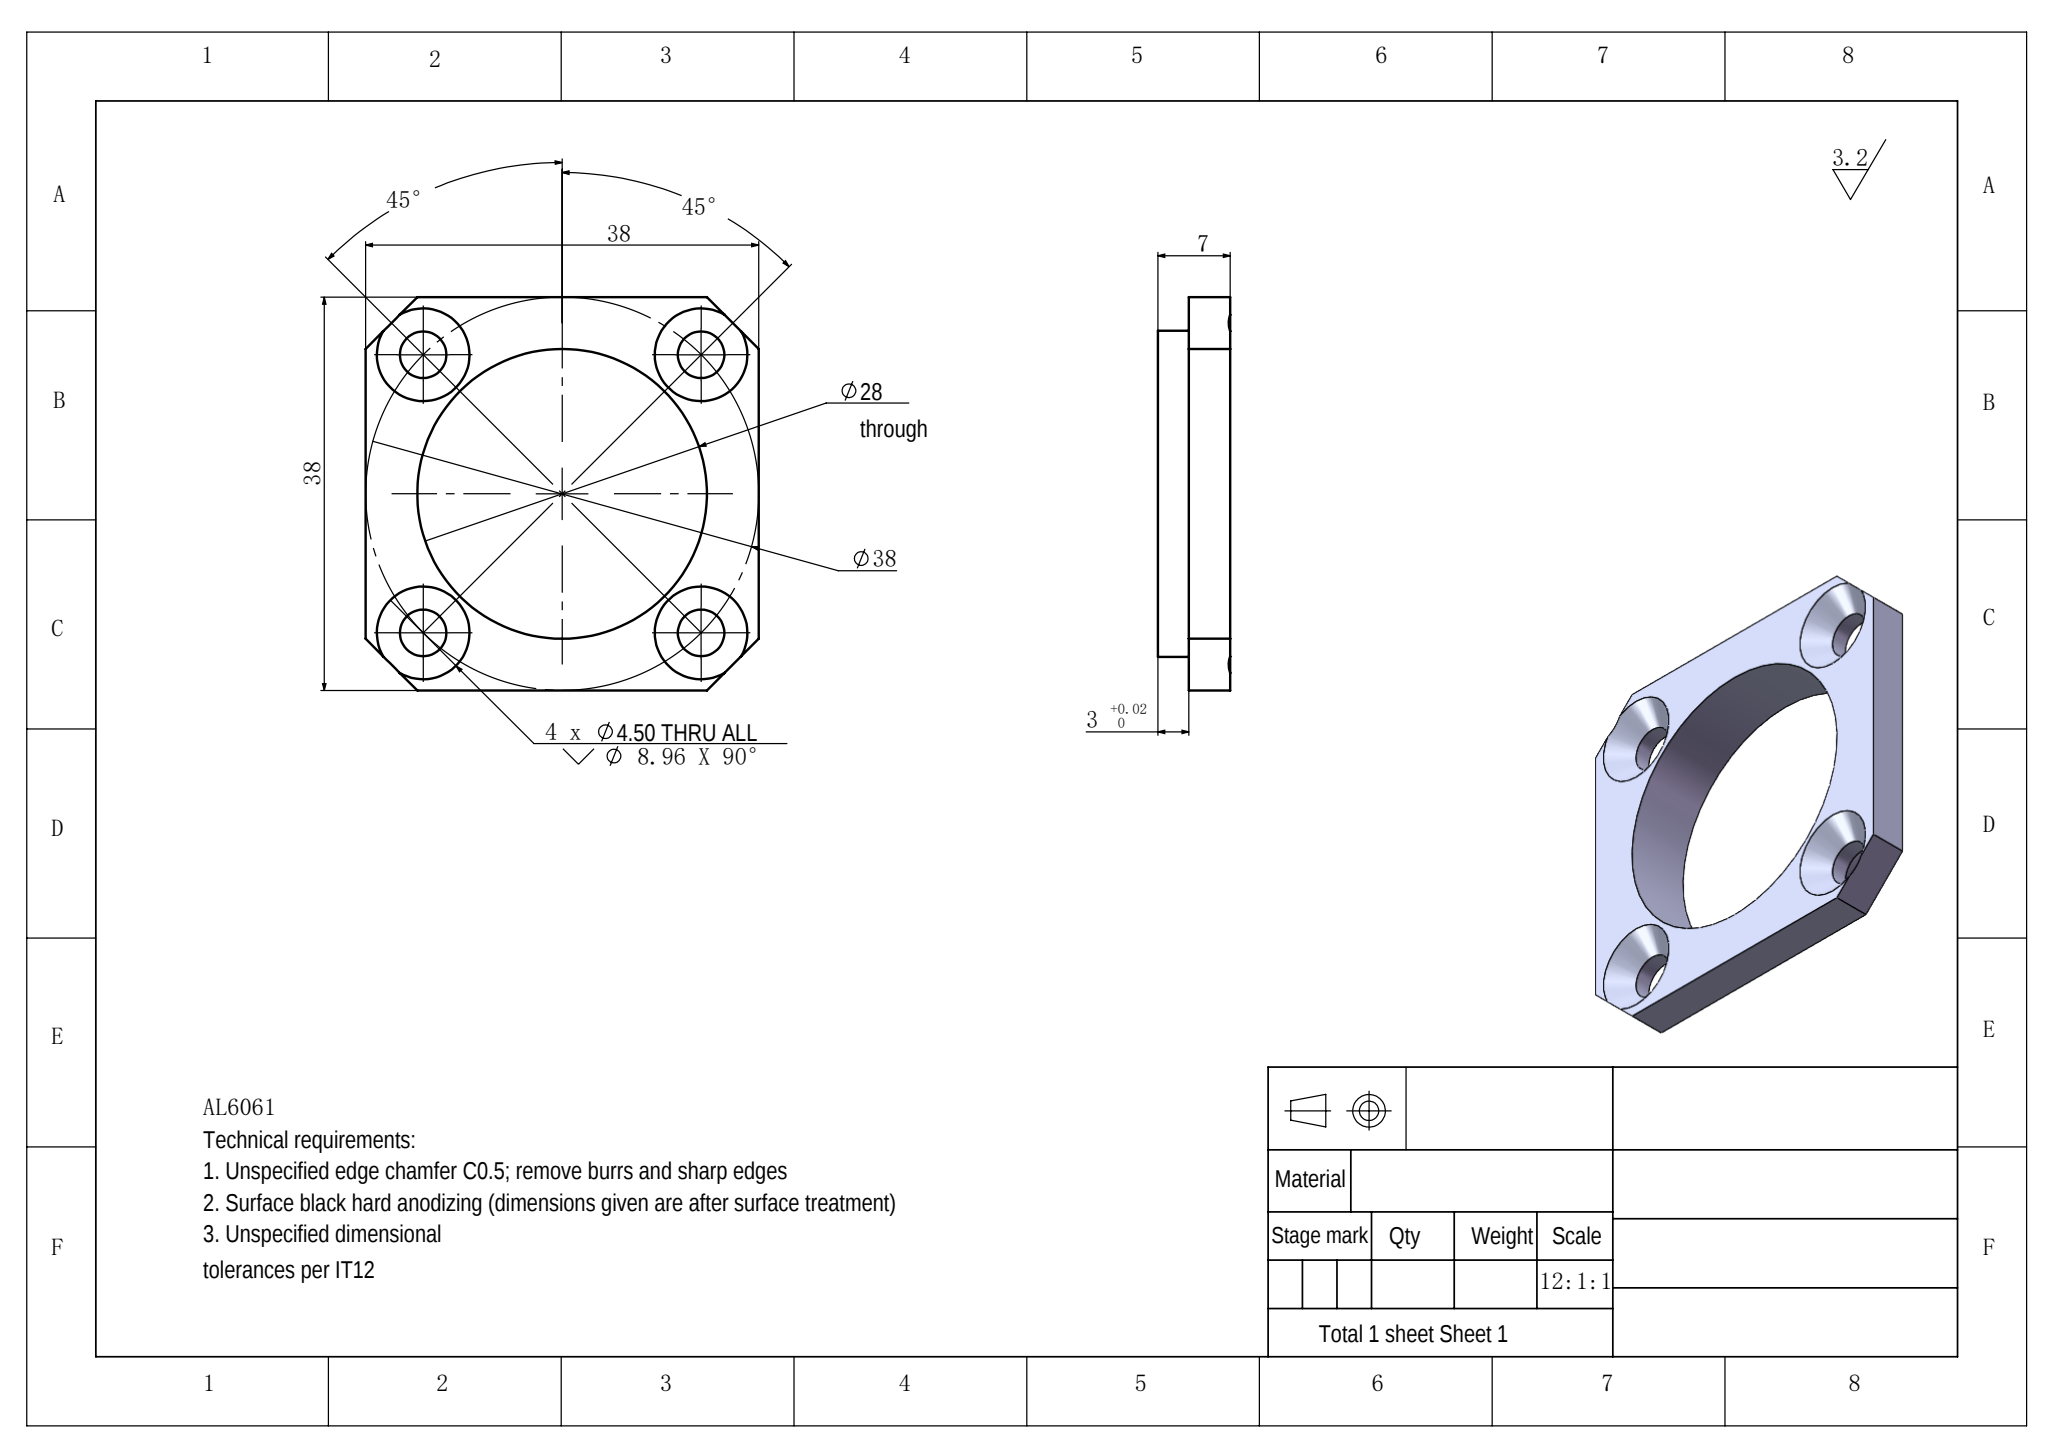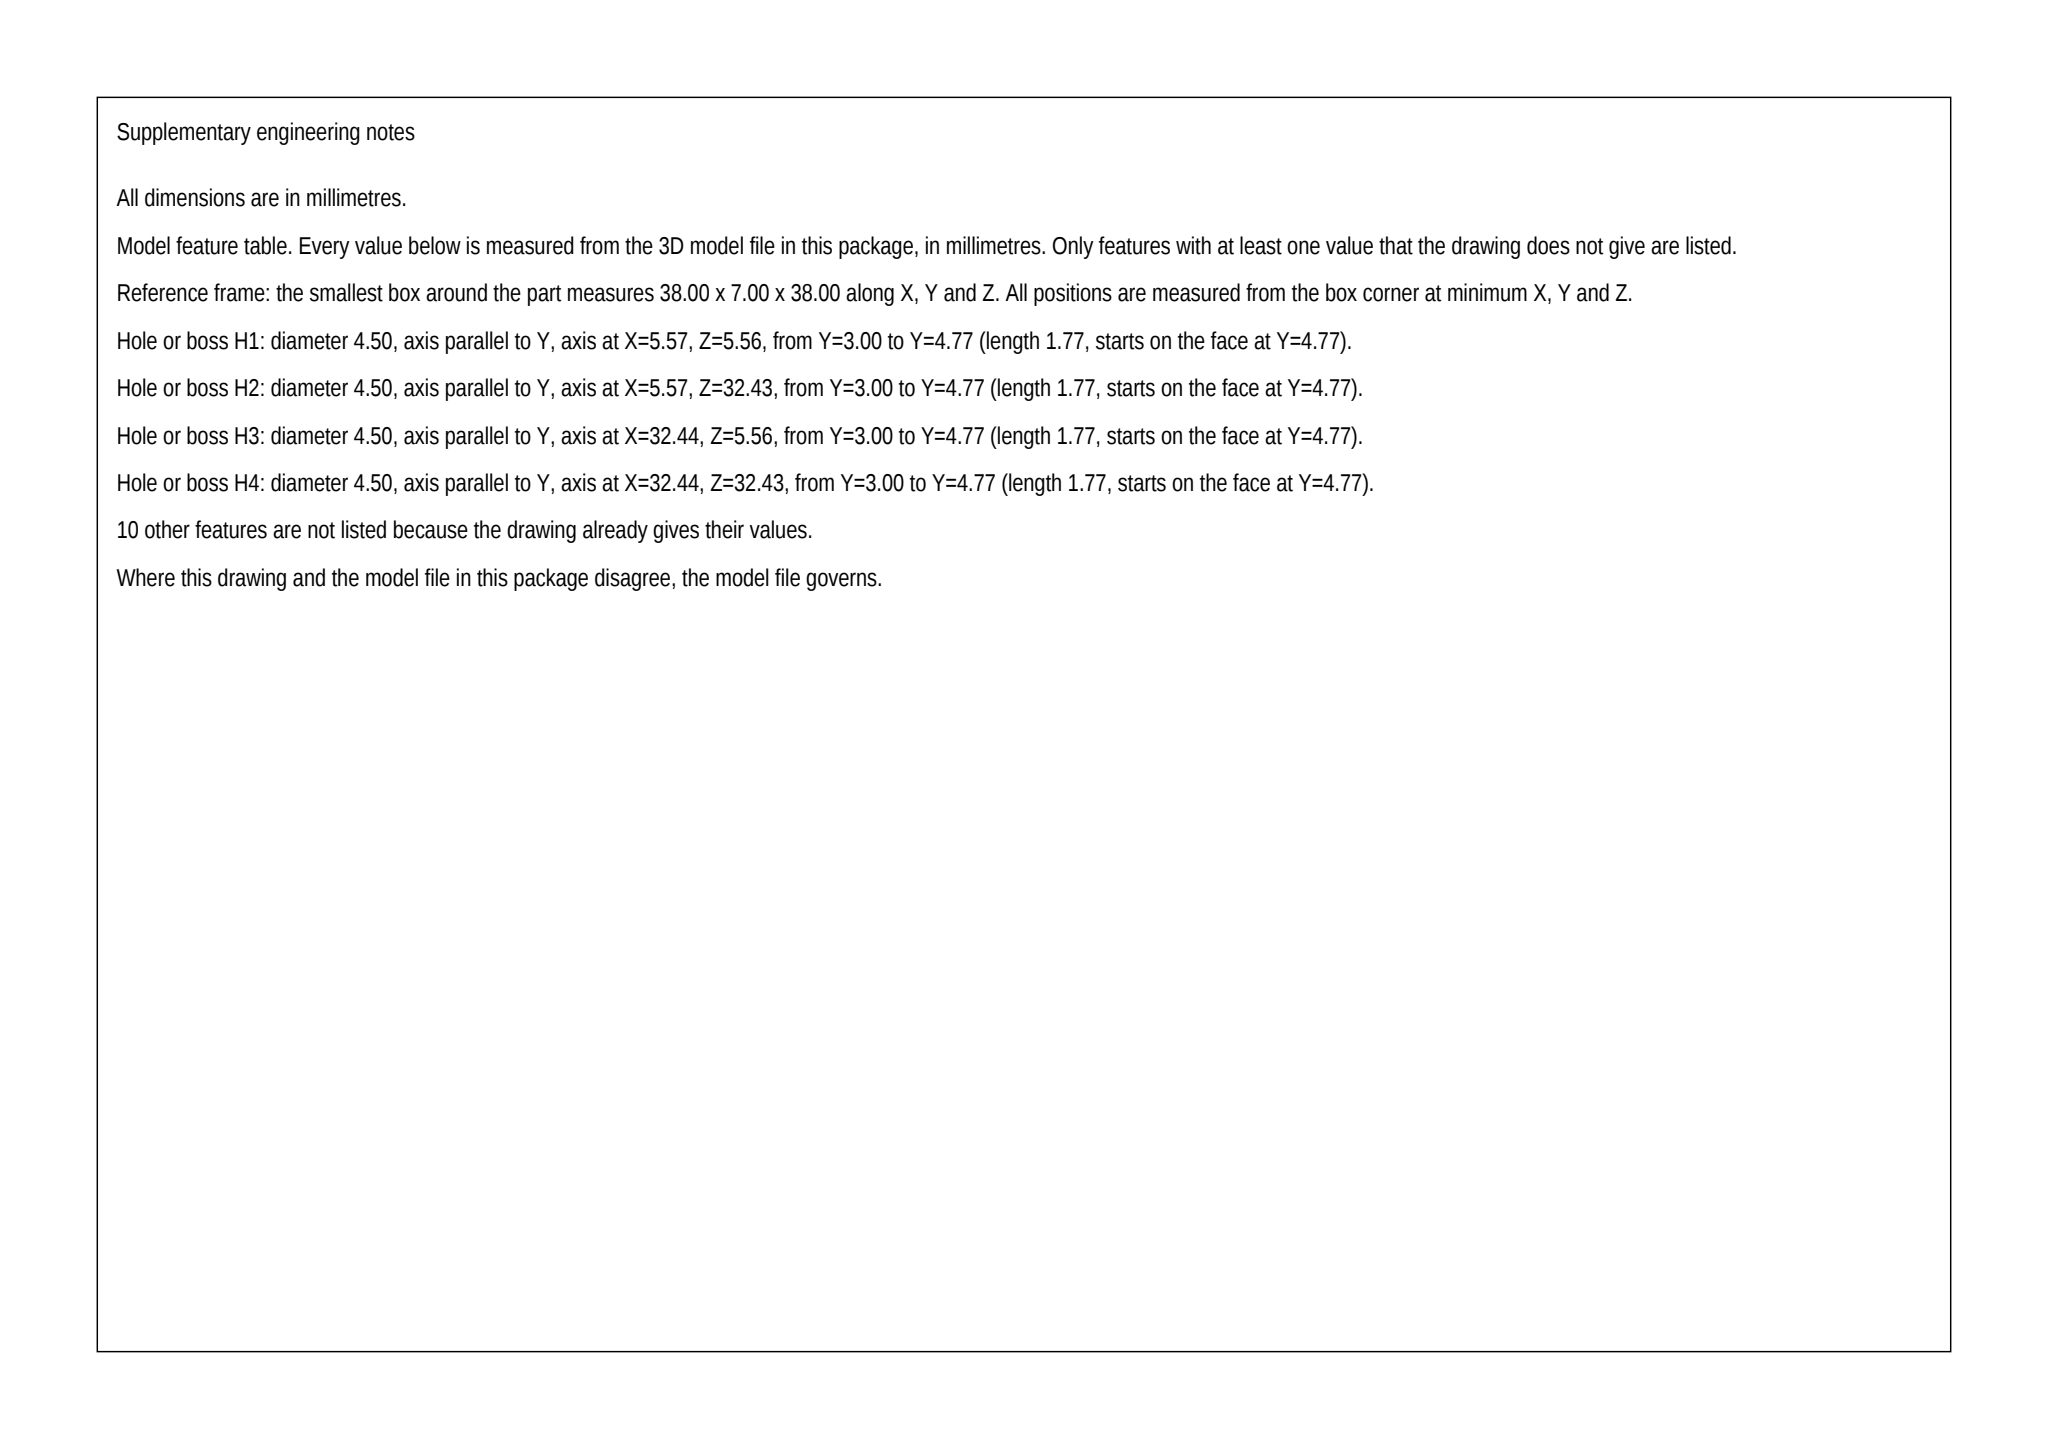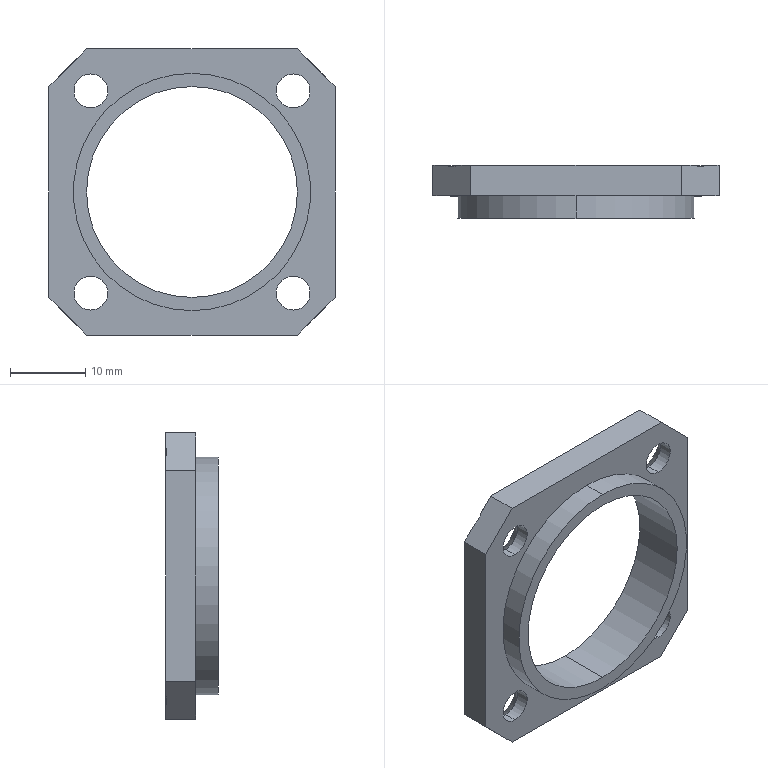Part | SolidWorks | mm | material AL6061 | 1 solid | 31 faces | box 38 x 7 x 38 mm | volume 3162 mm3 | cylinder 12 | plane 11 | cone 8 | commonest cylinder face diameters 4.5 x8 31.5 x2 28 x2
build123d program:
from build123d import *
from build123d.topology import SkipClean

# Parameters (mm, degrees)
SKETCH1_R                                    = 14
EXTRUDE1_DEPTH                               = 4
M4_HEX_SOCKET_COUNTERSUNK_HEAD_SCREW_2_COUNT = 2
M4_HEX_SOCKET_COUNTERSUNK_HEAD_SCREW_2_PITCH = 26.87
M4_HEX_SOCKET_COUNTERSUNK_HEAD_SCREW_3_COUNT = 2
M4_HEX_SOCKET_COUNTERSUNK_HEAD_SCREW_3_PITCH = 26.87
M4_HEX_SOCKET_COUNTERSUNK_HEAD_SCREW_4_COUNT = 2
M4_HEX_SOCKET_COUNTERSUNK_HEAD_SCREW_4_PITCH = 38
BOSS_EXTRUDE1_START                          = 3
SKETCH4_R                                    = 15.75
SKETCH4_R_2                                  = 14
BOSS_EXTRUDE1_DEPTH                          = 3


with BuildPart() as part:
    # Sketch1 → Extrude1 (new body)
    with BuildSketch(Plane(origin=(0, 0, 0), x_dir=(1, 0, 0), z_dir=(0, 1, 0))):
        Polygon((-81.535, -12.039), (-76.535, -7.039), (-48.535, -7.039), (-43.535, -12.039), (-43.535, -40.039), (-48.535, -45.039), (-76.535, -45.039), (-81.535, -40.039), align=None)
        with Locations(Location((-62.535, -26.039, 0), (0, 0, 270))):
            Circle(SKETCH1_R, mode=Mode.SUBTRACT)
    extrude(amount=EXTRUDE1_DEPTH)

    # Sketch3 → M4 Hex Socket Countersunk Head Screw Cou (revolve, cut)
    with BuildSketch(Plane(origin=(-75.97, 4, 12.604), x_dir=(0, 0, 1), z_dir=(1, 0, 0))):
        Polygon((0, 0), (0, 4), (2.25, 4), (2.25, 2.23), (4.48, 0), align=None)
    m4_hex_socket_countersunk_head_screw_cou = revolve(axis=Axis((-75.97, 10.35, 12.604), (0, -1, 0)), mode=Mode.SUBTRACT)

    # M4 Hex Socket Countersunk Head Screw 2: M4 Hex Socket Countersunk Head Screw Cou ×2
    with Locations(*[(i * M4_HEX_SOCKET_COUNTERSUNK_HEAD_SCREW_2_PITCH, 0, 0) for i in range(1, M4_HEX_SOCKET_COUNTERSUNK_HEAD_SCREW_2_COUNT)]):
        add(m4_hex_socket_countersunk_head_screw_cou, mode=Mode.SUBTRACT)

    # M4 Hex Socket Countersunk Head Screw 3: M4 Hex Socket Countersunk Head Screw Cou ×2
    with Locations(*[(0, 0, i * M4_HEX_SOCKET_COUNTERSUNK_HEAD_SCREW_3_PITCH) for i in range(1, M4_HEX_SOCKET_COUNTERSUNK_HEAD_SCREW_3_COUNT)]):
        add(m4_hex_socket_countersunk_head_screw_cou, mode=Mode.SUBTRACT)

    # M4 Hex Socket Countersunk Head Screw 4: M4 Hex Socket Countersunk Head Screw Cou ×2
    with Locations(*[Vector(0.7071, 0, 0.7071) * (i * M4_HEX_SOCKET_COUNTERSUNK_HEAD_SCREW_4_PITCH) for i in range(1, M4_HEX_SOCKET_COUNTERSUNK_HEAD_SCREW_4_COUNT)]):
        add(m4_hex_socket_countersunk_head_screw_cou, mode=Mode.SUBTRACT)

    # Sketch4 → Boss-Extrude1 (add)
    with SkipClean():  # the faces are left unmerged after this step: merging them gives an invalid solid
        with BuildSketch(Plane.XZ.offset(BOSS_EXTRUDE1_START)):
            with Locations(Location((-62.535, 26.039, 0), (0, 0, 270))):
                Circle(SKETCH4_R)
            with Locations(Location((-62.535, 26.039, 0), (0, 0, 270))):
                Circle(SKETCH4_R_2, mode=Mode.SUBTRACT)
        extrude(amount=-BOSS_EXTRUDE1_DEPTH)


solid = part.part